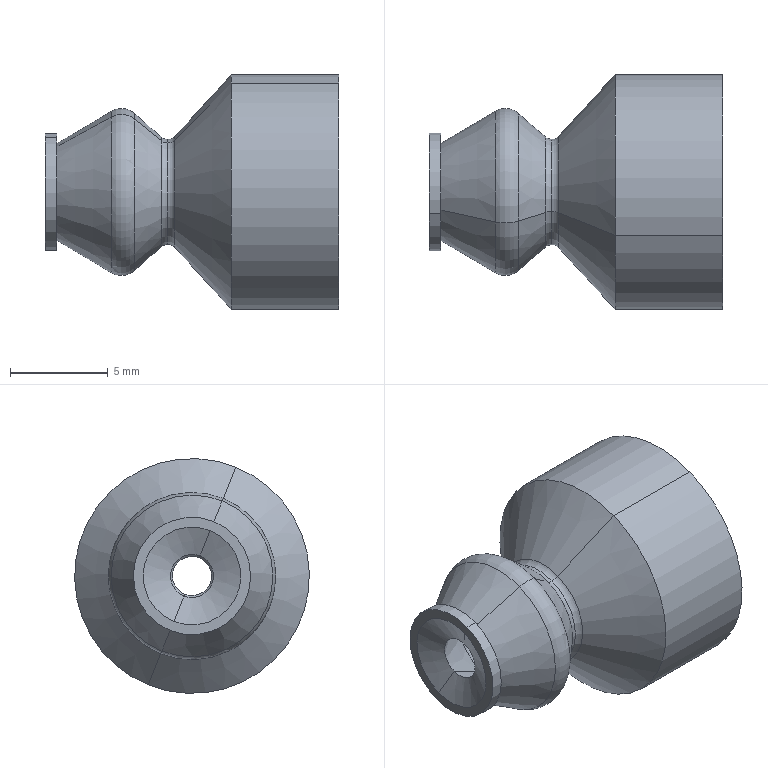Component | SolidWorks | VPDT6-1 | 1 solid | 37 faces | box 15 x 12 x 12 mm | volume 747 mm3 | cone 12 | torus 10 | cylinder 10 | plane 5 | commonest cylinder face diameters 7 x2 5 x2 12 x2 6 x2 2 x2
build123d program:
from build123d import *

# Parameters (mm, degrees)
SKETCH1_R                 = 3.5
SNAPCAVITYCLEARANCE_DEPTH = 0.7


with BuildPart() as part:
    # Sketch1_2 → Revolve1 (revolve)
    with BuildSketch(Plane.XY, mode=Mode.PRIVATE) as revolve1_sk:
        with BuildLine():
            Line((0, 15), (6, 15))
            Line((6, 15), (6, 9.5))
            Line((6, 9.5), (2.86, 6.629))
            ThreePointArc((2.86, 6.629), (2.698, 6.289), (2.82, 5.932))
            Line((2.82, 5.932), (4.028, 4.543))
            ThreePointArc((4.028, 4.543), (4.269, 3.979), (4.135, 3.38))
            Line((4.135, 3.38), (2.5, 0.6))
            Line((2.5, 0.6), (3, 0.6))
            Line((3, 0.6), (3, 0))
            Line((3, 0), (0, 0))
            Line((0, 0), (0, 15))
        make_face()
    revolve(revolve1_sk.sketch.rotate(Axis((0, 0, 0), (0, 1, 0)), 270), axis=Axis((0, 0, 0), (0, 1, 0)))

    # Sketch2 → Cut-Revolve1 (revolve, cut)
    with BuildSketch(Plane.XY, mode=Mode.PRIVATE) as cut_revolve1_sk:
        with BuildLine():
            Line((0, 15), (2.5, 15))
            Line((2.5, 15), (2.5, 12.5))
            Line((2.5, 12.5), (3.5, 12.5))
            ThreePointArc((3.5, 12.5), (4.5, 11.5), (3.5, 10.5))
            Line((3.5, 10.5), (1, 10.5))
            Line((1, 10.5), (1, 6.3))
            Line((1, 6.3), (2.841, 4.607))
            ThreePointArc((2.841, 4.607), (3.159, 3.967), (2.969, 3.278))
            Line((2.969, 3.278), (1.1, 0.6))
            Line((1.1, 0.6), (2.5, 0))
            Line((2.5, 0), (0, 0))
            Line((0, 0), (0, 15))
        make_face()
    revolve(cut_revolve1_sk.sketch.rotate(Axis((0, 0, 0), (0, 1, 0)), 270), axis=Axis((0, 0, 0), (0, 1, 0)), mode=Mode.SUBTRACT)

    # Sketch1 → SnapCavityClearance (cut)
    with BuildSketch(Plane(origin=(0, 10.5, 0), x_dir=(1, 0, 0), z_dir=(0, 1, 0))):
        with Locations(Location((0, 0, 0), (0, 0, 270))):
            Circle(SKETCH1_R)
    extrude(amount=-SNAPCAVITYCLEARANCE_DEPTH, mode=Mode.SUBTRACT)


solid = part.part

# Placed as in the assembly
solid = solid.moved(Location((-186.952, 37.141, -105.536), (0, 0, -90)))
STEP:
#1=COLOUR_RGB('',0.7922,0.8196,0.9333);
#2=FILL_AREA_STYLE_COLOUR('',#1);
#3=FILL_AREA_STYLE('',(#2));
#4=SURFACE_STYLE_FILL_AREA(#3);
#5=SURFACE_SIDE_STYLE('',(#4));
#6=SURFACE_STYLE_USAGE(.BOTH.,#5);
#7=PRESENTATION_STYLE_ASSIGNMENT((#6));
#8=CARTESIAN_POINT('',(-7.099,1.42,-4.05));
#9=VERTEX_POINT('',#8);
#10=CARTESIAN_POINT('',(-7.114,1.423,-4.056));
#11=VERTEX_POINT('',#10);
#12=CARTESIAN_POINT('',(-7.114,1.415,-4.038));
#13=DIRECTION('',(0.,0.9281,0.3723));
#14=DIRECTION('',(0.,-0.3723,0.9281));
#15=AXIS2_PLACEMENT_3D('',#12,#13,#14);
#16=CIRCLE('',#15,0.01969);
#17=EDGE_CURVE('',#9,#11,#16,.T.);
#18=ORIENTED_EDGE('',*,*,#17,.T.);
#19=CARTESIAN_POINT('',(-7.114,1.502,-4.254));
#20=VERTEX_POINT('',#19);
#21=CARTESIAN_POINT('',(-7.114,1.462,-4.155));
#22=DIRECTION('',(1.,-0.,-0.));
#23=DIRECTION('',(0.,1.,0.));
#24=AXIS2_PLACEMENT_3D('',#21,#22,#23);
#25=CIRCLE('',#24,0.1062);
#26=EDGE_CURVE('',#11,#20,#25,.T.);
#27=ORIENTED_EDGE('',*,*,#26,.T.);
#28=CARTESIAN_POINT('',(-7.099,1.504,-4.259));
#29=VERTEX_POINT('',#28);
#30=CARTESIAN_POINT('',(-7.114,1.509,-4.272));
#31=DIRECTION('',(-0.,-0.9281,-0.3723));
#32=DIRECTION('',(0.,0.3723,-0.9281));
#33=AXIS2_PLACEMENT_3D('',#30,#31,#32);
#34=CIRCLE('',#33,0.01969);
#35=EDGE_CURVE('',#29,#20,#34,.T.);
#36=ORIENTED_EDGE('',*,*,#35,.F.);
#37=CARTESIAN_POINT('',(-7.099,1.462,-4.155));
#38=DIRECTION('',(1.,-0.,-0.));
#39=DIRECTION('',(0.,-0.3723,0.9281));
#40=AXIS2_PLACEMENT_3D('',#37,#38,#39);
#41=CIRCLE('',#40,0.1126);
#42=EDGE_CURVE('',#9,#29,#41,.T.);
#43=ORIENTED_EDGE('',*,*,#42,.F.);
#44=EDGE_LOOP('',(#18,#27,#36,#43));
#45=FACE_OUTER_BOUND('',#44,.T.);
#46=CARTESIAN_POINT('',(-7.114,1.462,-4.155));
#47=DIRECTION('',(1.,-0.,-0.));
#48=DIRECTION('',(-0.,-0.3723,0.9281));
#49=AXIS2_PLACEMENT_3D('',#46,#47,#48);
#50=TOROIDAL_SURFACE('',#49,0.1259,0.01969);
#51=ADVANCED_FACE('',(#45),#50,.F.);
#52=ORIENTED_EDGE('',*,*,#35,.T.);
#53=CARTESIAN_POINT('',(-7.114,1.462,-4.155));
#54=DIRECTION('',(1.,-0.,-0.));
#55=DIRECTION('',(0.,1.,0.));
#56=AXIS2_PLACEMENT_3D('',#53,#54,#55);
#57=CIRCLE('',#56,0.1062);
#58=EDGE_CURVE('',#20,#11,#57,.T.);
#59=ORIENTED_EDGE('',*,*,#58,.T.);
#60=ORIENTED_EDGE('',*,*,#17,.F.);
#61=CARTESIAN_POINT('',(-7.099,1.462,-4.155));
#62=DIRECTION('',(1.,-0.,-0.));
#63=DIRECTION('',(0.,-0.3723,0.9281));
#64=AXIS2_PLACEMENT_3D('',#61,#62,#63);
#65=CIRCLE('',#64,0.1126);
#66=EDGE_CURVE('',#29,#9,#65,.T.);
#67=ORIENTED_EDGE('',*,*,#66,.F.);
#68=EDGE_LOOP('',(#52,#59,#60,#67));
#69=FACE_OUTER_BOUND('',#68,.T.);
#70=CARTESIAN_POINT('',(-7.114,1.462,-4.155));
#71=DIRECTION('',(1.,-0.,-0.));
#72=DIRECTION('',(-0.,-0.3723,0.9281));
#73=AXIS2_PLACEMENT_3D('',#70,#71,#72);
#74=TOROIDAL_SURFACE('',#73,0.1259,0.01969);
#75=ADVANCED_FACE('',(#69),#74,.F.);
#76=CARTESIAN_POINT('',(-6.974,1.514,-4.283));
#77=VERTEX_POINT('',#76);
#78=CARTESIAN_POINT('',(-6.974,1.411,-4.027));
#79=VERTEX_POINT('',#78);
#80=CARTESIAN_POINT('',(-6.974,1.462,-4.155));
#81=DIRECTION('',(1.,-0.,-0.));
#82=DIRECTION('',(0.,-0.3723,0.9281));
#83=AXIS2_PLACEMENT_3D('',#80,#81,#82);
#84=CIRCLE('',#83,0.1378);
#85=EDGE_CURVE('',#77,#79,#84,.T.);
#86=ORIENTED_EDGE('',*,*,#85,.F.);
#87=CARTESIAN_POINT('',(-6.947,1.514,-4.283));
#88=VERTEX_POINT('',#87);
#89=CARTESIAN_POINT('',(-6.974,1.514,-4.283));
#90=DIRECTION('',(1.,-0.,-0.));
#91=VECTOR('',#90,39.37);
#92=LINE('',#89,#91);
#93=EDGE_CURVE('',#77,#88,#92,.T.);
#94=ORIENTED_EDGE('',*,*,#93,.T.);
#95=CARTESIAN_POINT('',(-6.947,1.411,-4.027));
#96=VERTEX_POINT('',#95);
#97=CARTESIAN_POINT('',(-6.947,1.462,-4.155));
#98=DIRECTION('',(1.,-0.,-0.));
#99=DIRECTION('',(0.,-0.3723,0.9281));
#100=AXIS2_PLACEMENT_3D('',#97,#98,#99);
#101=CIRCLE('',#100,0.1378);
#102=EDGE_CURVE('',#88,#96,#101,.T.);
#103=ORIENTED_EDGE('',*,*,#102,.T.);
#104=CARTESIAN_POINT('',(-6.974,1.411,-4.027));
#105=DIRECTION('',(1.,-0.,-0.));
#106=VECTOR('',#105,39.37);
#107=LINE('',#104,#106);
#108=EDGE_CURVE('',#79,#96,#107,.T.);
#109=ORIENTED_EDGE('',*,*,#108,.F.);
#110=EDGE_LOOP('',(#86,#94,#103,#109));
#111=FACE_OUTER_BOUND('',#110,.T.);
#112=CARTESIAN_POINT('',(-6.974,1.462,-4.155));
#113=DIRECTION('',(1.,-0.,-0.));
#114=DIRECTION('',(0.,-0.3723,0.9281));
#115=AXIS2_PLACEMENT_3D('',#112,#113,#114);
#116=CYLINDRICAL_SURFACE('',#115,0.1378);
#117=ADVANCED_FACE('',(#111),#116,.F.);
#118=CARTESIAN_POINT('',(-7.337,1.478,-4.195));
#119=VERTEX_POINT('',#118);
#120=CARTESIAN_POINT('',(-7.337,1.446,-4.115));
#121=VERTEX_POINT('',#120);
#122=CARTESIAN_POINT('',(-7.337,1.462,-4.155));
#123=DIRECTION('',(1.,-0.,-0.));
#124=DIRECTION('',(0.,-0.3723,0.9281));
#125=AXIS2_PLACEMENT_3D('',#122,#123,#124);
#126=CIRCLE('',#125,0.04331);
#127=EDGE_CURVE('',#119,#121,#126,.T.);
#128=ORIENTED_EDGE('',*,*,#127,.T.);
#129=CARTESIAN_POINT('',(-7.36,1.426,-4.064));
#130=VERTEX_POINT('',#129);
#131=CARTESIAN_POINT('',(-7.36,1.426,-4.064));
#132=DIRECTION('',(-0.3939,-0.3422,0.8531));
#133=VECTOR('',#132,39.37);
#134=LINE('',#131,#133);
#135=EDGE_CURVE('',#121,#130,#134,.T.);
#136=ORIENTED_EDGE('',*,*,#135,.T.);
#137=CARTESIAN_POINT('',(-7.36,1.499,-4.246));
#138=VERTEX_POINT('',#137);
#139=CARTESIAN_POINT('',(-7.36,1.462,-4.155));
#140=DIRECTION('',(1.,-0.,-0.));
#141=DIRECTION('',(0.,-0.3723,0.9281));
#142=AXIS2_PLACEMENT_3D('',#139,#140,#141);
#143=CIRCLE('',#142,0.09843);
#144=EDGE_CURVE('',#138,#130,#143,.T.);
#145=ORIENTED_EDGE('',*,*,#144,.F.);
#146=CARTESIAN_POINT('',(-7.36,1.499,-4.246));
#147=DIRECTION('',(-0.3939,0.3422,-0.8531));
#148=VECTOR('',#147,39.37);
#149=LINE('',#146,#148);
#150=EDGE_CURVE('',#119,#138,#149,.T.);
#151=ORIENTED_EDGE('',*,*,#150,.F.);
#152=EDGE_LOOP('',(#128,#136,#145,#151));
#153=FACE_OUTER_BOUND('',#152,.T.);
#154=CARTESIAN_POINT('',(-7.36,1.462,-4.155));
#155=DIRECTION('',(-1.,0.,0.));
#156=DIRECTION('',(0.,0.3723,-0.9281));
#157=AXIS2_PLACEMENT_3D('',#154,#155,#156);
#158=CONICAL_SURFACE('',#157,0.09843,1.166);
#159=ADVANCED_FACE('',(#153),#158,.F.);
#160=ORIENTED_EDGE('',*,*,#127,.F.);
#161=CARTESIAN_POINT('',(-7.231,1.506,-4.263));
#162=VERTEX_POINT('',#161);
#163=CARTESIAN_POINT('',(-7.337,1.478,-4.195));
#164=DIRECTION('',(0.82,0.2131,-0.5312));
#165=VECTOR('',#164,39.37);
#166=LINE('',#163,#165);
#167=EDGE_CURVE('',#119,#162,#166,.T.);
#168=ORIENTED_EDGE('',*,*,#167,.T.);
#169=CARTESIAN_POINT('',(-7.231,1.419,-4.046));
#170=VERTEX_POINT('',#169);
#171=CARTESIAN_POINT('',(-7.231,1.462,-4.155));
#172=DIRECTION('',(1.,-0.,-0.));
#173=DIRECTION('',(0.,-0.3723,0.9281));
#174=AXIS2_PLACEMENT_3D('',#171,#172,#173);
#175=CIRCLE('',#174,0.1169);
#176=EDGE_CURVE('',#162,#170,#175,.T.);
#177=ORIENTED_EDGE('',*,*,#176,.T.);
#178=CARTESIAN_POINT('',(-7.337,1.446,-4.115));
#179=DIRECTION('',(0.82,-0.2131,0.5312));
#180=VECTOR('',#179,39.37);
#181=LINE('',#178,#180);
#182=EDGE_CURVE('',#121,#170,#181,.T.);
#183=ORIENTED_EDGE('',*,*,#182,.F.);
#184=EDGE_LOOP('',(#160,#168,#177,#183));
#185=FACE_OUTER_BOUND('',#184,.T.);
#186=CARTESIAN_POINT('',(-7.337,1.462,-4.155));
#187=DIRECTION('',(1.,-0.,-0.));
#188=DIRECTION('',(0.,-0.3723,0.9281));
#189=AXIS2_PLACEMENT_3D('',#186,#187,#188);
#190=CONICAL_SURFACE('',#189,0.04331,0.6094);
#191=ADVANCED_FACE('',(#185),#190,.F.);
#192=ORIENTED_EDGE('',*,*,#176,.F.);
#193=CARTESIAN_POINT('',(-7.179,1.504,-4.259));
#194=VERTEX_POINT('',#193);
#195=CARTESIAN_POINT('',(-7.208,1.494,-4.234));
#196=DIRECTION('',(-0.,-0.9281,-0.3723));
#197=DIRECTION('',(0.,0.3723,-0.9281));
#198=AXIS2_PLACEMENT_3D('',#195,#196,#197);
#199=CIRCLE('',#198,0.03937);
#200=EDGE_CURVE('',#162,#194,#199,.T.);
#201=ORIENTED_EDGE('',*,*,#200,.T.);
#202=CARTESIAN_POINT('',(-7.179,1.421,-4.051));
#203=VERTEX_POINT('',#202);
#204=CARTESIAN_POINT('',(-7.179,1.462,-4.155));
#205=DIRECTION('',(1.,-0.,-0.));
#206=DIRECTION('',(0.,-0.3723,0.9281));
#207=AXIS2_PLACEMENT_3D('',#204,#205,#206);
#208=CIRCLE('',#207,0.1118);
#209=EDGE_CURVE('',#194,#203,#208,.T.);
#210=ORIENTED_EDGE('',*,*,#209,.T.);
#211=CARTESIAN_POINT('',(-7.208,1.431,-4.076));
#212=DIRECTION('',(0.,0.9281,0.3723));
#213=DIRECTION('',(0.,-0.3723,0.9281));
#214=AXIS2_PLACEMENT_3D('',#211,#212,#213);
#215=CIRCLE('',#214,0.03937);
#216=EDGE_CURVE('',#170,#203,#215,.T.);
#217=ORIENTED_EDGE('',*,*,#216,.F.);
#218=EDGE_LOOP('',(#192,#201,#210,#217));
#219=FACE_OUTER_BOUND('',#218,.T.);
#220=CARTESIAN_POINT('',(-7.208,1.462,-4.155));
#221=DIRECTION('',(1.,-0.,-0.));
#222=DIRECTION('',(-0.,-0.3723,0.9281));
#223=AXIS2_PLACEMENT_3D('',#220,#221,#222);
#224=TOROIDAL_SURFACE('',#223,0.08518,0.03937);
#225=ADVANCED_FACE('',(#219),#224,.F.);
#226=CARTESIAN_POINT('',(-7.112,1.477,-4.192));
#227=VERTEX_POINT('',#226);
#228=CARTESIAN_POINT('',(-7.112,1.448,-4.118));
#229=VERTEX_POINT('',#228);
#230=CARTESIAN_POINT('',(-7.112,1.462,-4.155));
#231=DIRECTION('',(1.,-0.,-0.));
#232=DIRECTION('',(0.,-0.3723,0.9281));
#233=AXIS2_PLACEMENT_3D('',#230,#231,#232);
#234=CIRCLE('',#233,0.03937);
#235=EDGE_CURVE('',#227,#229,#234,.T.);
#236=ORIENTED_EDGE('',*,*,#235,.T.);
#237=CARTESIAN_POINT('',(-7.179,1.421,-4.051));
#238=DIRECTION('',(-0.6771,-0.274,0.683));
#239=VECTOR('',#238,39.37);
#240=LINE('',#237,#239);
#241=EDGE_CURVE('',#229,#203,#240,.T.);
#242=ORIENTED_EDGE('',*,*,#241,.T.);
#243=ORIENTED_EDGE('',*,*,#209,.F.);
#244=CARTESIAN_POINT('',(-7.179,1.504,-4.259));
#245=DIRECTION('',(-0.6771,0.274,-0.683));
#246=VECTOR('',#245,39.37);
#247=LINE('',#244,#246);
#248=EDGE_CURVE('',#227,#194,#247,.T.);
#249=ORIENTED_EDGE('',*,*,#248,.F.);
#250=EDGE_LOOP('',(#236,#242,#243,#249));
#251=FACE_OUTER_BOUND('',#250,.T.);
#252=CARTESIAN_POINT('',(-7.179,1.462,-4.155));
#253=DIRECTION('',(-1.,0.,0.));
#254=DIRECTION('',(0.,0.3723,-0.9281));
#255=AXIS2_PLACEMENT_3D('',#252,#253,#254);
#256=CONICAL_SURFACE('',#255,0.1118,0.827);
#257=ADVANCED_FACE('',(#251),#256,.F.);
#258=ORIENTED_EDGE('',*,*,#102,.F.);
#259=CARTESIAN_POINT('',(-6.868,1.514,-4.283));
#260=VERTEX_POINT('',#259);
#261=CARTESIAN_POINT('',(-6.908,1.514,-4.283));
#262=DIRECTION('',(-0.,-0.9281,-0.3723));
#263=DIRECTION('',(0.,0.3723,-0.9281));
#264=AXIS2_PLACEMENT_3D('',#261,#262,#263);
#265=CIRCLE('',#264,0.03937);
#266=EDGE_CURVE('',#88,#260,#265,.T.);
#267=ORIENTED_EDGE('',*,*,#266,.T.);
#268=CARTESIAN_POINT('',(-6.868,1.411,-4.027));
#269=VERTEX_POINT('',#268);
#270=CARTESIAN_POINT('',(-6.868,1.462,-4.155));
#271=DIRECTION('',(1.,-0.,-0.));
#272=DIRECTION('',(0.,-0.3723,0.9281));
#273=AXIS2_PLACEMENT_3D('',#270,#271,#272);
#274=CIRCLE('',#273,0.1378);
#275=EDGE_CURVE('',#260,#269,#274,.T.);
#276=ORIENTED_EDGE('',*,*,#275,.T.);
#277=CARTESIAN_POINT('',(-6.908,1.411,-4.027));
#278=DIRECTION('',(0.,0.9281,0.3723));
#279=DIRECTION('',(0.,-0.3723,0.9281));
#280=AXIS2_PLACEMENT_3D('',#277,#278,#279);
#281=CIRCLE('',#280,0.03937);
#282=EDGE_CURVE('',#96,#269,#281,.T.);
#283=ORIENTED_EDGE('',*,*,#282,.F.);
#284=EDGE_LOOP('',(#258,#267,#276,#283));
#285=FACE_OUTER_BOUND('',#284,.T.);
#286=CARTESIAN_POINT('',(-6.908,1.462,-4.155));
#287=DIRECTION('',(1.,-0.,-0.));
#288=DIRECTION('',(-0.,-0.3723,0.9281));
#289=AXIS2_PLACEMENT_3D('',#286,#287,#288);
#290=TOROIDAL_SURFACE('',#289,0.1378,0.03937);
#291=ADVANCED_FACE('',(#285),#290,.F.);
#292=CARTESIAN_POINT('',(-6.868,1.499,-4.246));
#293=VERTEX_POINT('',#292);
#294=CARTESIAN_POINT('',(-6.868,1.426,-4.064));
#295=VERTEX_POINT('',#294);
#296=CARTESIAN_POINT('',(-6.868,1.462,-4.155));
#297=DIRECTION('',(1.,-0.,-0.));
#298=DIRECTION('',(0.,-0.3723,0.9281));
#299=AXIS2_PLACEMENT_3D('',#296,#297,#298);
#300=CIRCLE('',#299,0.09843);
#301=EDGE_CURVE('',#293,#295,#300,.T.);
#302=ORIENTED_EDGE('',*,*,#301,.F.);
#303=CARTESIAN_POINT('',(-6.77,1.499,-4.246));
#304=VERTEX_POINT('',#303);
#305=CARTESIAN_POINT('',(-7.36,1.499,-4.246));
#306=DIRECTION('',(1.,-0.,-0.));
#307=VECTOR('',#306,39.37);
#308=LINE('',#305,#307);
#309=EDGE_CURVE('',#293,#304,#308,.T.);
#310=ORIENTED_EDGE('',*,*,#309,.T.);
#311=CARTESIAN_POINT('',(-6.77,1.426,-4.064));
#312=VERTEX_POINT('',#311);
#313=CARTESIAN_POINT('',(-6.77,1.462,-4.155));
#314=DIRECTION('',(1.,-0.,-0.));
#315=DIRECTION('',(0.,-0.3723,0.9281));
#316=AXIS2_PLACEMENT_3D('',#313,#314,#315);
#317=CIRCLE('',#316,0.09843);
#318=EDGE_CURVE('',#304,#312,#317,.T.);
#319=ORIENTED_EDGE('',*,*,#318,.T.);
#320=CARTESIAN_POINT('',(-7.36,1.426,-4.064));
#321=DIRECTION('',(1.,-0.,-0.));
#322=VECTOR('',#321,39.37);
#323=LINE('',#320,#322);
#324=EDGE_CURVE('',#295,#312,#323,.T.);
#325=ORIENTED_EDGE('',*,*,#324,.F.);
#326=EDGE_LOOP('',(#302,#310,#319,#325));
#327=FACE_OUTER_BOUND('',#326,.T.);
#328=CARTESIAN_POINT('',(-7.36,1.462,-4.155));
#329=DIRECTION('',(1.,-0.,-0.));
#330=DIRECTION('',(0.,-0.3723,0.9281));
#331=AXIS2_PLACEMENT_3D('',#328,#329,#330);
#332=CYLINDRICAL_SURFACE('',#331,0.09843);
#333=ADVANCED_FACE('',(#327),#332,.F.);
#334=CARTESIAN_POINT('',(-6.986,1.374,-3.936));
#335=VERTEX_POINT('',#334);
#336=CARTESIAN_POINT('',(-6.986,1.55,-4.374));
#337=VERTEX_POINT('',#336);
#338=CARTESIAN_POINT('',(-6.986,1.462,-4.155));
#339=DIRECTION('',(1.,-0.,-0.));
#340=DIRECTION('',(0.,-0.3723,0.9281));
#341=AXIS2_PLACEMENT_3D('',#338,#339,#340);
#342=CIRCLE('',#341,0.2362);
#343=EDGE_CURVE('',#335,#337,#342,.T.);
#344=ORIENTED_EDGE('',*,*,#343,.T.);
#345=CARTESIAN_POINT('',(-6.77,1.55,-4.374));
#346=VERTEX_POINT('',#345);
#347=CARTESIAN_POINT('',(-7.36,1.55,-4.374));
#348=DIRECTION('',(1.,-0.,-0.));
#349=VECTOR('',#348,39.37);
#350=LINE('',#347,#349);
#351=EDGE_CURVE('',#337,#346,#350,.T.);
#352=ORIENTED_EDGE('',*,*,#351,.T.);
#353=CARTESIAN_POINT('',(-6.77,1.374,-3.936));
#354=VERTEX_POINT('',#353);
#355=CARTESIAN_POINT('',(-6.77,1.462,-4.155));
#356=DIRECTION('',(1.,-0.,-0.));
#357=DIRECTION('',(0.,-0.3723,0.9281));
#358=AXIS2_PLACEMENT_3D('',#355,#356,#357);
#359=CIRCLE('',#358,0.2362);
#360=EDGE_CURVE('',#354,#346,#359,.T.);
#361=ORIENTED_EDGE('',*,*,#360,.F.);
#362=CARTESIAN_POINT('',(-7.36,1.374,-3.936));
#363=DIRECTION('',(1.,-0.,-0.));
#364=VECTOR('',#363,39.37);
#365=LINE('',#362,#364);
#366=EDGE_CURVE('',#335,#354,#365,.T.);
#367=ORIENTED_EDGE('',*,*,#366,.F.);
#368=EDGE_LOOP('',(#344,#352,#361,#367));
#369=FACE_OUTER_BOUND('',#368,.T.);
#370=CARTESIAN_POINT('',(-7.36,1.462,-4.155));
#371=DIRECTION('',(1.,-0.,-0.));
#372=DIRECTION('',(0.,-0.3723,0.9281));
#373=AXIS2_PLACEMENT_3D('',#370,#371,#372);
#374=CYLINDRICAL_SURFACE('',#373,0.2362);
#375=ADVANCED_FACE('',(#369),#374,.T.);
#376=ORIENTED_EDGE('',*,*,#42,.T.);
#377=CARTESIAN_POINT('',(-7.099,1.504,-4.259));
#378=DIRECTION('',(0.6748,0.2748,-0.685));
#379=VECTOR('',#378,39.37);
#380=LINE('',#377,#379);
#381=EDGE_CURVE('',#29,#337,#380,.T.);
#382=ORIENTED_EDGE('',*,*,#381,.T.);
#383=ORIENTED_EDGE('',*,*,#343,.F.);
#384=CARTESIAN_POINT('',(-7.099,1.42,-4.05));
#385=DIRECTION('',(0.6748,-0.2748,0.685));
#386=VECTOR('',#385,39.37);
#387=LINE('',#384,#386);
#388=EDGE_CURVE('',#9,#335,#387,.T.);
#389=ORIENTED_EDGE('',*,*,#388,.F.);
#390=EDGE_LOOP('',(#376,#382,#383,#389));
#391=FACE_OUTER_BOUND('',#390,.T.);
#392=CARTESIAN_POINT('',(-7.099,1.462,-4.155));
#393=DIRECTION('',(1.,-0.,-0.));
#394=DIRECTION('',(0.,-0.3723,0.9281));
#395=AXIS2_PLACEMENT_3D('',#392,#393,#394);
#396=CONICAL_SURFACE('',#395,0.1126,0.8301);
#397=ADVANCED_FACE('',(#391),#396,.T.);
#398=ORIENTED_EDGE('',*,*,#58,.F.);
#399=CARTESIAN_POINT('',(-7.127,1.504,-4.258));
#400=VERTEX_POINT('',#399);
#401=CARTESIAN_POINT('',(-7.114,1.509,-4.272));
#402=DIRECTION('',(-0.,-0.9281,-0.3723));
#403=DIRECTION('',(0.,0.3723,-0.9281));
#404=AXIS2_PLACEMENT_3D('',#401,#402,#403);
#405=CIRCLE('',#404,0.01969);
#406=EDGE_CURVE('',#20,#400,#405,.T.);
#407=ORIENTED_EDGE('',*,*,#406,.T.);
#408=CARTESIAN_POINT('',(-7.127,1.421,-4.052));
#409=VERTEX_POINT('',#408);
#410=CARTESIAN_POINT('',(-7.127,1.462,-4.155));
#411=DIRECTION('',(1.,-0.,-0.));
#412=DIRECTION('',(0.,-0.3723,0.9281));
#413=AXIS2_PLACEMENT_3D('',#410,#411,#412);
#414=CIRCLE('',#413,0.111);
#415=EDGE_CURVE('',#400,#409,#414,.T.);
#416=ORIENTED_EDGE('',*,*,#415,.T.);
#417=CARTESIAN_POINT('',(-7.114,1.415,-4.038));
#418=DIRECTION('',(0.,0.9281,0.3723));
#419=DIRECTION('',(0.,-0.3723,0.9281));
#420=AXIS2_PLACEMENT_3D('',#417,#418,#419);
#421=CIRCLE('',#420,0.01969);
#422=EDGE_CURVE('',#11,#409,#421,.T.);
#423=ORIENTED_EDGE('',*,*,#422,.F.);
#424=EDGE_LOOP('',(#398,#407,#416,#423));
#425=FACE_OUTER_BOUND('',#424,.T.);
#426=CARTESIAN_POINT('',(-7.114,1.462,-4.155));
#427=DIRECTION('',(1.,-0.,-0.));
#428=DIRECTION('',(-0.,-0.3723,0.9281));
#429=AXIS2_PLACEMENT_3D('',#426,#427,#428);
#430=TOROIDAL_SURFACE('',#429,0.1259,0.01969);
#431=ADVANCED_FACE('',(#425),#430,.F.);
#432=CARTESIAN_POINT('',(-7.127,1.462,-4.155));
#433=DIRECTION('',(1.,-0.,-0.));
#434=DIRECTION('',(0.,-0.3723,0.9281));
#435=AXIS2_PLACEMENT_3D('',#432,#433,#434);
#436=CIRCLE('',#435,0.111);
#437=EDGE_CURVE('',#409,#400,#436,.T.);
#438=ORIENTED_EDGE('',*,*,#437,.F.);
#439=CARTESIAN_POINT('',(-7.181,1.403,-4.008));
#440=VERTEX_POINT('',#439);
#441=CARTESIAN_POINT('',(-7.181,1.403,-4.008));
#442=DIRECTION('',(-0.7546,-0.2443,0.609));
#443=VECTOR('',#442,39.37);
#444=LINE('',#441,#443);
#445=EDGE_CURVE('',#409,#440,#444,.T.);
#446=ORIENTED_EDGE('',*,*,#445,.T.);
#447=CARTESIAN_POINT('',(-7.181,1.521,-4.302));
#448=VERTEX_POINT('',#447);
#449=CARTESIAN_POINT('',(-7.181,1.462,-4.155));
#450=DIRECTION('',(1.,-0.,-0.));
#451=DIRECTION('',(0.,-0.3723,0.9281));
#452=AXIS2_PLACEMENT_3D('',#449,#450,#451);
#453=CIRCLE('',#452,0.1586);
#454=EDGE_CURVE('',#440,#448,#453,.T.);
#455=ORIENTED_EDGE('',*,*,#454,.T.);
#456=CARTESIAN_POINT('',(-7.181,1.521,-4.302));
#457=DIRECTION('',(-0.7546,0.2443,-0.609));
#458=VECTOR('',#457,39.37);
#459=LINE('',#456,#458);
#460=EDGE_CURVE('',#400,#448,#459,.T.);
#461=ORIENTED_EDGE('',*,*,#460,.F.);
#462=EDGE_LOOP('',(#438,#446,#455,#461));
#463=FACE_OUTER_BOUND('',#462,.T.);
#464=CARTESIAN_POINT('',(-7.181,1.462,-4.155));
#465=DIRECTION('',(-1.,0.,0.));
#466=DIRECTION('',(0.,0.3723,-0.9281));
#467=AXIS2_PLACEMENT_3D('',#464,#465,#466);
#468=CONICAL_SURFACE('',#467,0.1586,0.7157);
#469=ADVANCED_FACE('',(#463),#468,.T.);
#470=CARTESIAN_POINT('',(-7.227,1.402,-4.004));
#471=VERTEX_POINT('',#470);
#472=CARTESIAN_POINT('',(-7.227,1.523,-4.306));
#473=VERTEX_POINT('',#472);
#474=CARTESIAN_POINT('',(-7.227,1.462,-4.155));
#475=DIRECTION('',(1.,-0.,-0.));
#476=DIRECTION('',(0.,-0.3723,0.9281));
#477=AXIS2_PLACEMENT_3D('',#474,#475,#476);
#478=CIRCLE('',#477,0.1628);
#479=EDGE_CURVE('',#471,#473,#478,.T.);
#480=ORIENTED_EDGE('',*,*,#479,.T.);
#481=CARTESIAN_POINT('',(-7.207,1.51,-4.275));
#482=DIRECTION('',(-0.,-0.9281,-0.3723));
#483=DIRECTION('',(0.,0.3723,-0.9281));
#484=AXIS2_PLACEMENT_3D('',#481,#482,#483);
#485=CIRCLE('',#484,0.03937);
#486=EDGE_CURVE('',#473,#448,#485,.T.);
#487=ORIENTED_EDGE('',*,*,#486,.T.);
#488=ORIENTED_EDGE('',*,*,#454,.F.);
#489=CARTESIAN_POINT('',(-7.207,1.414,-4.035));
#490=DIRECTION('',(0.,0.9281,0.3723));
#491=DIRECTION('',(0.,-0.3723,0.9281));
#492=AXIS2_PLACEMENT_3D('',#489,#490,#491);
#493=CIRCLE('',#492,0.03937);
#494=EDGE_CURVE('',#471,#440,#493,.T.);
#495=ORIENTED_EDGE('',*,*,#494,.F.);
#496=EDGE_LOOP('',(#480,#487,#488,#495));
#497=FACE_OUTER_BOUND('',#496,.T.);
#498=CARTESIAN_POINT('',(-7.207,1.462,-4.155));
#499=DIRECTION('',(1.,-0.,-0.));
#500=DIRECTION('',(-0.,-0.3723,0.9281));
#501=AXIS2_PLACEMENT_3D('',#498,#499,#500);
#502=TOROIDAL_SURFACE('',#501,0.1289,0.03937);
#503=ADVANCED_FACE('',(#497),#502,.T.);
#504=CARTESIAN_POINT('',(-7.337,1.426,-4.064));
#505=VERTEX_POINT('',#504);
#506=CARTESIAN_POINT('',(-7.337,1.499,-4.246));
#507=VERTEX_POINT('',#506);
#508=CARTESIAN_POINT('',(-7.337,1.462,-4.155));
#509=DIRECTION('',(1.,-0.,-0.));
#510=DIRECTION('',(0.,-0.3723,0.9281));
#511=AXIS2_PLACEMENT_3D('',#508,#509,#510);
#512=CIRCLE('',#511,0.09843);
#513=EDGE_CURVE('',#505,#507,#512,.T.);
#514=ORIENTED_EDGE('',*,*,#513,.T.);
#515=CARTESIAN_POINT('',(-7.337,1.499,-4.246));
#516=DIRECTION('',(0.8619,0.1888,-0.4706));
#517=VECTOR('',#516,39.37);
#518=LINE('',#515,#517);
#519=EDGE_CURVE('',#507,#473,#518,.T.);
#520=ORIENTED_EDGE('',*,*,#519,.T.);
#521=ORIENTED_EDGE('',*,*,#479,.F.);
#522=CARTESIAN_POINT('',(-7.337,1.426,-4.064));
#523=DIRECTION('',(0.8619,-0.1888,0.4706));
#524=VECTOR('',#523,39.37);
#525=LINE('',#522,#524);
#526=EDGE_CURVE('',#505,#471,#525,.T.);
#527=ORIENTED_EDGE('',*,*,#526,.F.);
#528=EDGE_LOOP('',(#514,#520,#521,#527));
#529=FACE_OUTER_BOUND('',#528,.T.);
#530=CARTESIAN_POINT('',(-7.337,1.462,-4.155));
#531=DIRECTION('',(1.,-0.,-0.));
#532=DIRECTION('',(0.,-0.3723,0.9281));
#533=AXIS2_PLACEMENT_3D('',#530,#531,#532);
#534=CONICAL_SURFACE('',#533,0.09843,0.5317);
#535=ADVANCED_FACE('',(#529),#534,.T.);
#536=CARTESIAN_POINT('',(-7.36,1.418,-4.045));
#537=VERTEX_POINT('',#536);
#538=CARTESIAN_POINT('',(-7.36,1.506,-4.265));
#539=VERTEX_POINT('',#538);
#540=CARTESIAN_POINT('',(-7.36,1.462,-4.155));
#541=DIRECTION('',(1.,-0.,-0.));
#542=DIRECTION('',(0.,-0.3723,0.9281));
#543=AXIS2_PLACEMENT_3D('',#540,#541,#542);
#544=CIRCLE('',#543,0.1181);
#545=EDGE_CURVE('',#537,#539,#544,.T.);
#546=ORIENTED_EDGE('',*,*,#545,.T.);
#547=CARTESIAN_POINT('',(-7.337,1.506,-4.265));
#548=VERTEX_POINT('',#547);
#549=CARTESIAN_POINT('',(-7.36,1.506,-4.265));
#550=DIRECTION('',(1.,-0.,-0.));
#551=VECTOR('',#550,39.37);
#552=LINE('',#549,#551);
#553=EDGE_CURVE('',#539,#548,#552,.T.);
#554=ORIENTED_EDGE('',*,*,#553,.T.);
#555=CARTESIAN_POINT('',(-7.337,1.418,-4.045));
#556=VERTEX_POINT('',#555);
#557=CARTESIAN_POINT('',(-7.337,1.462,-4.155));
#558=DIRECTION('',(1.,-0.,-0.));
#559=DIRECTION('',(0.,-0.3723,0.9281));
#560=AXIS2_PLACEMENT_3D('',#557,#558,#559);
#561=CIRCLE('',#560,0.1181);
#562=EDGE_CURVE('',#556,#548,#561,.T.);
#563=ORIENTED_EDGE('',*,*,#562,.F.);
#564=CARTESIAN_POINT('',(-7.36,1.418,-4.045));
#565=DIRECTION('',(1.,-0.,-0.));
#566=VECTOR('',#565,39.37);
#567=LINE('',#564,#566);
#568=EDGE_CURVE('',#537,#556,#567,.T.);
#569=ORIENTED_EDGE('',*,*,#568,.F.);
#570=EDGE_LOOP('',(#546,#554,#563,#569));
#571=FACE_OUTER_BOUND('',#570,.T.);
#572=CARTESIAN_POINT('',(-7.36,1.462,-4.155));
#573=DIRECTION('',(1.,-0.,-0.));
#574=DIRECTION('',(0.,-0.3723,0.9281));
#575=AXIS2_PLACEMENT_3D('',#572,#573,#574);
#576=CYLINDRICAL_SURFACE('',#575,0.1181);
#577=ADVANCED_FACE('',(#571),#576,.T.);
#578=ORIENTED_EDGE('',*,*,#235,.F.);
#579=CARTESIAN_POINT('',(-6.974,1.477,-4.192));
#580=VERTEX_POINT('',#579);
#581=CARTESIAN_POINT('',(-7.36,1.477,-4.192));
#582=DIRECTION('',(1.,-0.,-0.));
#583=VECTOR('',#582,39.37);
#584=LINE('',#581,#583);
#585=EDGE_CURVE('',#227,#580,#584,.T.);
#586=ORIENTED_EDGE('',*,*,#585,.T.);
#587=CARTESIAN_POINT('',(-6.974,1.448,-4.118));
#588=VERTEX_POINT('',#587);
#589=CARTESIAN_POINT('',(-6.974,1.462,-4.155));
#590=DIRECTION('',(1.,-0.,-0.));
#591=DIRECTION('',(0.,-0.3723,0.9281));
#592=AXIS2_PLACEMENT_3D('',#589,#590,#591);
#593=CIRCLE('',#592,0.03937);
#594=EDGE_CURVE('',#580,#588,#593,.T.);
#595=ORIENTED_EDGE('',*,*,#594,.T.);
#596=CARTESIAN_POINT('',(-7.36,1.448,-4.118));
#597=DIRECTION('',(1.,-0.,-0.));
#598=VECTOR('',#597,39.37);
#599=LINE('',#596,#598);
#600=EDGE_CURVE('',#229,#588,#599,.T.);
#601=ORIENTED_EDGE('',*,*,#600,.F.);
#602=EDGE_LOOP('',(#578,#586,#595,#601));
#603=FACE_OUTER_BOUND('',#602,.T.);
#604=CARTESIAN_POINT('',(-7.36,1.462,-4.155));
#605=DIRECTION('',(1.,-0.,-0.));
#606=DIRECTION('',(0.,-0.3723,0.9281));
#607=AXIS2_PLACEMENT_3D('',#604,#605,#606);
#608=CYLINDRICAL_SURFACE('',#607,0.03937);
#609=ADVANCED_FACE('',(#603),#608,.F.);
#610=ORIENTED_EDGE('',*,*,#585,.F.);
#611=CARTESIAN_POINT('',(-7.112,1.462,-4.155));
#612=DIRECTION('',(1.,-0.,-0.));
#613=DIRECTION('',(0.,-0.3723,0.9281));
#614=AXIS2_PLACEMENT_3D('',#611,#612,#613);
#615=CIRCLE('',#614,0.03937);
#616=EDGE_CURVE('',#229,#227,#615,.T.);
#617=ORIENTED_EDGE('',*,*,#616,.F.);
#618=ORIENTED_EDGE('',*,*,#600,.T.);
#619=CARTESIAN_POINT('',(-6.974,1.462,-4.155));
#620=DIRECTION('',(1.,-0.,-0.));
#621=DIRECTION('',(0.,-0.3723,0.9281));
#622=AXIS2_PLACEMENT_3D('',#619,#620,#621);
#623=CIRCLE('',#622,0.03937);
#624=EDGE_CURVE('',#588,#580,#623,.T.);
#625=ORIENTED_EDGE('',*,*,#624,.T.);
#626=EDGE_LOOP('',(#610,#617,#618,#625));
#627=FACE_OUTER_BOUND('',#626,.T.);
#628=CARTESIAN_POINT('',(-7.36,1.462,-4.155));
#629=DIRECTION('',(1.,-0.,-0.));
#630=DIRECTION('',(0.,-0.3723,0.9281));
#631=AXIS2_PLACEMENT_3D('',#628,#629,#630);
#632=CYLINDRICAL_SURFACE('',#631,0.03937);
#633=ADVANCED_FACE('',(#627),#632,.F.);
#634=ORIENTED_EDGE('',*,*,#545,.F.);
#635=CARTESIAN_POINT('',(-7.36,1.462,-4.155));
#636=DIRECTION('',(1.,-0.,-0.));
#637=DIRECTION('',(0.,-0.3723,0.9281));
#638=AXIS2_PLACEMENT_3D('',#635,#636,#637);
#639=CIRCLE('',#638,0.1181);
#640=EDGE_CURVE('',#539,#537,#639,.T.);
#641=ORIENTED_EDGE('',*,*,#640,.F.);
#642=EDGE_LOOP('',(#634,#641));
#643=FACE_OUTER_BOUND('',#642,.T.);
#644=ORIENTED_EDGE('',*,*,#144,.T.);
#645=CARTESIAN_POINT('',(-7.36,1.462,-4.155));
#646=DIRECTION('',(1.,-0.,-0.));
#647=DIRECTION('',(0.,-0.3723,0.9281));
#648=AXIS2_PLACEMENT_3D('',#645,#646,#647);
#649=CIRCLE('',#648,0.09843);
#650=EDGE_CURVE('',#130,#138,#649,.T.);
#651=ORIENTED_EDGE('',*,*,#650,.T.);
#652=EDGE_LOOP('',(#644,#651));
#653=FACE_BOUND('',#652,.T.);
#654=CARTESIAN_POINT('',(-7.36,1.353,-4.199));
#655=DIRECTION('',(1.,-0.,-0.));
#656=DIRECTION('',(-0.,-0.3723,0.9281));
#657=AXIS2_PLACEMENT_3D('',#654,#655,#656);
#658=PLANE('',#657);
#659=ADVANCED_FACE('',(#643,#653),#658,.F.);
#660=ORIENTED_EDGE('',*,*,#360,.T.);
#661=CARTESIAN_POINT('',(-6.77,1.462,-4.155));
#662=DIRECTION('',(1.,-0.,-0.));
#663=DIRECTION('',(0.,-0.3723,0.9281));
#664=AXIS2_PLACEMENT_3D('',#661,#662,#663);
#665=CIRCLE('',#664,0.2362);
#666=EDGE_CURVE('',#346,#354,#665,.T.);
#667=ORIENTED_EDGE('',*,*,#666,.T.);
#668=EDGE_LOOP('',(#660,#667));
#669=FACE_OUTER_BOUND('',#668,.T.);
#670=CARTESIAN_POINT('',(-6.77,1.462,-4.155));
#671=DIRECTION('',(1.,-0.,-0.));
#672=DIRECTION('',(0.,-0.3723,0.9281));
#673=AXIS2_PLACEMENT_3D('',#670,#671,#672);
#674=CIRCLE('',#673,0.09843);
#675=EDGE_CURVE('',#312,#304,#674,.T.);
#676=ORIENTED_EDGE('',*,*,#675,.F.);
#677=ORIENTED_EDGE('',*,*,#318,.F.);
#678=EDGE_LOOP('',(#676,#677));
#679=FACE_BOUND('',#678,.T.);
#680=CARTESIAN_POINT('',(-6.77,1.462,-4.155));
#681=DIRECTION('',(-1.,0.,0.));
#682=DIRECTION('',(0.,0.3723,-0.9281));
#683=AXIS2_PLACEMENT_3D('',#680,#681,#682);
#684=PLANE('',#683);
#685=ADVANCED_FACE('',(#669,#679),#684,.F.);
#686=ORIENTED_EDGE('',*,*,#553,.F.);
#687=ORIENTED_EDGE('',*,*,#640,.T.);
#688=ORIENTED_EDGE('',*,*,#568,.T.);
#689=CARTESIAN_POINT('',(-7.337,1.462,-4.155));
#690=DIRECTION('',(1.,-0.,-0.));
#691=DIRECTION('',(0.,-0.3723,0.9281));
#692=AXIS2_PLACEMENT_3D('',#689,#690,#691);
#693=CIRCLE('',#692,0.1181);
#694=EDGE_CURVE('',#548,#556,#693,.T.);
#695=ORIENTED_EDGE('',*,*,#694,.F.);
#696=EDGE_LOOP('',(#686,#687,#688,#695));
#697=FACE_OUTER_BOUND('',#696,.T.);
#698=CARTESIAN_POINT('',(-7.36,1.462,-4.155));
#699=DIRECTION('',(1.,-0.,-0.));
#700=DIRECTION('',(0.,-0.3723,0.9281));
#701=AXIS2_PLACEMENT_3D('',#698,#699,#700);
#702=CYLINDRICAL_SURFACE('',#701,0.1181);
#703=ADVANCED_FACE('',(#697),#702,.T.);
#704=ORIENTED_EDGE('',*,*,#513,.F.);
#705=CARTESIAN_POINT('',(-7.337,1.462,-4.155));
#706=DIRECTION('',(1.,-0.,-0.));
#707=DIRECTION('',(0.,-0.3723,0.9281));
#708=AXIS2_PLACEMENT_3D('',#705,#706,#707);
#709=CIRCLE('',#708,0.09843);
#710=EDGE_CURVE('',#507,#505,#709,.T.);
#711=ORIENTED_EDGE('',*,*,#710,.F.);
#712=EDGE_LOOP('',(#704,#711));
#713=FACE_BOUND('',#712,.T.);
#714=ORIENTED_EDGE('',*,*,#562,.T.);
#715=ORIENTED_EDGE('',*,*,#694,.T.);
#716=EDGE_LOOP('',(#714,#715));
#717=FACE_OUTER_BOUND('',#716,.T.);
#718=CARTESIAN_POINT('',(-7.337,1.371,-4.192));
#719=DIRECTION('',(-1.,0.,0.));
#720=DIRECTION('',(0.,0.3723,-0.9281));
#721=AXIS2_PLACEMENT_3D('',#718,#719,#720);
#722=PLANE('',#721);
#723=ADVANCED_FACE('',(#713,#717),#722,.F.);
#724=ORIENTED_EDGE('',*,*,#519,.F.);
#725=ORIENTED_EDGE('',*,*,#710,.T.);
#726=ORIENTED_EDGE('',*,*,#526,.T.);
#727=CARTESIAN_POINT('',(-7.227,1.462,-4.155));
#728=DIRECTION('',(1.,-0.,-0.));
#729=DIRECTION('',(0.,-0.3723,0.9281));
#730=AXIS2_PLACEMENT_3D('',#727,#728,#729);
#731=CIRCLE('',#730,0.1628);
#732=EDGE_CURVE('',#473,#471,#731,.T.);
#733=ORIENTED_EDGE('',*,*,#732,.F.);
#734=EDGE_LOOP('',(#724,#725,#726,#733));
#735=FACE_OUTER_BOUND('',#734,.T.);
#736=CARTESIAN_POINT('',(-7.337,1.462,-4.155));
#737=DIRECTION('',(1.,-0.,-0.));
#738=DIRECTION('',(0.,-0.3723,0.9281));
#739=AXIS2_PLACEMENT_3D('',#736,#737,#738);
#740=CONICAL_SURFACE('',#739,0.09843,0.5317);
#741=ADVANCED_FACE('',(#735),#740,.T.);
#742=ORIENTED_EDGE('',*,*,#486,.F.);
#743=ORIENTED_EDGE('',*,*,#732,.T.);
#744=ORIENTED_EDGE('',*,*,#494,.T.);
#745=CARTESIAN_POINT('',(-7.181,1.462,-4.155));
#746=DIRECTION('',(1.,-0.,-0.));
#747=DIRECTION('',(0.,-0.3723,0.9281));
#748=AXIS2_PLACEMENT_3D('',#745,#746,#747);
#749=CIRCLE('',#748,0.1586);
#750=EDGE_CURVE('',#448,#440,#749,.T.);
#751=ORIENTED_EDGE('',*,*,#750,.F.);
#752=EDGE_LOOP('',(#742,#743,#744,#751));
#753=FACE_OUTER_BOUND('',#752,.T.);
#754=CARTESIAN_POINT('',(-7.207,1.462,-4.155));
#755=DIRECTION('',(1.,-0.,-0.));
#756=DIRECTION('',(-0.,-0.3723,0.9281));
#757=AXIS2_PLACEMENT_3D('',#754,#755,#756);
#758=TOROIDAL_SURFACE('',#757,0.1289,0.03937);
#759=ADVANCED_FACE('',(#753),#758,.T.);
#760=ORIENTED_EDGE('',*,*,#445,.F.);
#761=ORIENTED_EDGE('',*,*,#415,.F.);
#762=ORIENTED_EDGE('',*,*,#460,.T.);
#763=ORIENTED_EDGE('',*,*,#750,.T.);
#764=EDGE_LOOP('',(#760,#761,#762,#763));
#765=FACE_OUTER_BOUND('',#764,.T.);
#766=CARTESIAN_POINT('',(-7.181,1.462,-4.155));
#767=DIRECTION('',(-1.,0.,0.));
#768=DIRECTION('',(0.,0.3723,-0.9281));
#769=AXIS2_PLACEMENT_3D('',#766,#767,#768);
#770=CONICAL_SURFACE('',#769,0.1586,0.7157);
#771=ADVANCED_FACE('',(#765),#770,.T.);
#772=ORIENTED_EDGE('',*,*,#26,.F.);
#773=ORIENTED_EDGE('',*,*,#422,.T.);
#774=ORIENTED_EDGE('',*,*,#437,.T.);
#775=ORIENTED_EDGE('',*,*,#406,.F.);
#776=EDGE_LOOP('',(#772,#773,#774,#775));
#777=FACE_OUTER_BOUND('',#776,.T.);
#778=CARTESIAN_POINT('',(-7.114,1.462,-4.155));
#779=DIRECTION('',(1.,-0.,-0.));
#780=DIRECTION('',(-0.,-0.3723,0.9281));
#781=AXIS2_PLACEMENT_3D('',#778,#779,#780);
#782=TOROIDAL_SURFACE('',#781,0.1259,0.01969);
#783=ADVANCED_FACE('',(#777),#782,.F.);
#784=ORIENTED_EDGE('',*,*,#381,.F.);
#785=ORIENTED_EDGE('',*,*,#66,.T.);
#786=ORIENTED_EDGE('',*,*,#388,.T.);
#787=CARTESIAN_POINT('',(-6.986,1.462,-4.155));
#788=DIRECTION('',(1.,-0.,-0.));
#789=DIRECTION('',(0.,-0.3723,0.9281));
#790=AXIS2_PLACEMENT_3D('',#787,#788,#789);
#791=CIRCLE('',#790,0.2362);
#792=EDGE_CURVE('',#337,#335,#791,.T.);
#793=ORIENTED_EDGE('',*,*,#792,.F.);
#794=EDGE_LOOP('',(#784,#785,#786,#793));
#795=FACE_OUTER_BOUND('',#794,.T.);
#796=CARTESIAN_POINT('',(-7.099,1.462,-4.155));
#797=DIRECTION('',(1.,-0.,-0.));
#798=DIRECTION('',(0.,-0.3723,0.9281));
#799=AXIS2_PLACEMENT_3D('',#796,#797,#798);
#800=CONICAL_SURFACE('',#799,0.1126,0.8301);
#801=ADVANCED_FACE('',(#795),#800,.T.);
#802=ORIENTED_EDGE('',*,*,#351,.F.);
#803=ORIENTED_EDGE('',*,*,#792,.T.);
#804=ORIENTED_EDGE('',*,*,#366,.T.);
#805=ORIENTED_EDGE('',*,*,#666,.F.);
#806=EDGE_LOOP('',(#802,#803,#804,#805));
#807=FACE_OUTER_BOUND('',#806,.T.);
#808=CARTESIAN_POINT('',(-7.36,1.462,-4.155));
#809=DIRECTION('',(1.,-0.,-0.));
#810=DIRECTION('',(0.,-0.3723,0.9281));
#811=AXIS2_PLACEMENT_3D('',#808,#809,#810);
#812=CYLINDRICAL_SURFACE('',#811,0.2362);
#813=ADVANCED_FACE('',(#807),#812,.T.);
#814=ORIENTED_EDGE('',*,*,#309,.F.);
#815=CARTESIAN_POINT('',(-6.868,1.462,-4.155));
#816=DIRECTION('',(1.,-0.,-0.));
#817=DIRECTION('',(0.,-0.3723,0.9281));
#818=AXIS2_PLACEMENT_3D('',#815,#816,#817);
#819=CIRCLE('',#818,0.09843);
#820=EDGE_CURVE('',#295,#293,#819,.T.);
#821=ORIENTED_EDGE('',*,*,#820,.F.);
#822=ORIENTED_EDGE('',*,*,#324,.T.);
#823=ORIENTED_EDGE('',*,*,#675,.T.);
#824=EDGE_LOOP('',(#814,#821,#822,#823));
#825=FACE_OUTER_BOUND('',#824,.T.);
#826=CARTESIAN_POINT('',(-7.36,1.462,-4.155));
#827=DIRECTION('',(1.,-0.,-0.));
#828=DIRECTION('',(0.,-0.3723,0.9281));
#829=AXIS2_PLACEMENT_3D('',#826,#827,#828);
#830=CYLINDRICAL_SURFACE('',#829,0.09843);
#831=ADVANCED_FACE('',(#825),#830,.F.);
#832=ORIENTED_EDGE('',*,*,#820,.T.);
#833=ORIENTED_EDGE('',*,*,#301,.T.);
#834=EDGE_LOOP('',(#832,#833));
#835=FACE_BOUND('',#834,.T.);
#836=CARTESIAN_POINT('',(-6.868,1.462,-4.155));
#837=DIRECTION('',(1.,-0.,-0.));
#838=DIRECTION('',(0.,-0.3723,0.9281));
#839=AXIS2_PLACEMENT_3D('',#836,#837,#838);
#840=CIRCLE('',#839,0.1378);
#841=EDGE_CURVE('',#269,#260,#840,.T.);
#842=ORIENTED_EDGE('',*,*,#841,.F.);
#843=ORIENTED_EDGE('',*,*,#275,.F.);
#844=EDGE_LOOP('',(#842,#843));
#845=FACE_OUTER_BOUND('',#844,.T.);
#846=CARTESIAN_POINT('',(-6.868,1.371,-4.192));
#847=DIRECTION('',(-1.,0.,0.));
#848=DIRECTION('',(0.,0.3723,-0.9281));
#849=AXIS2_PLACEMENT_3D('',#846,#847,#848);
#850=PLANE('',#849);
#851=ADVANCED_FACE('',(#835,#845),#850,.T.);
#852=ORIENTED_EDGE('',*,*,#266,.F.);
#853=CARTESIAN_POINT('',(-6.947,1.462,-4.155));
#854=DIRECTION('',(1.,-0.,-0.));
#855=DIRECTION('',(0.,-0.3723,0.9281));
#856=AXIS2_PLACEMENT_3D('',#853,#854,#855);
#857=CIRCLE('',#856,0.1378);
#858=EDGE_CURVE('',#96,#88,#857,.T.);
#859=ORIENTED_EDGE('',*,*,#858,.F.);
#860=ORIENTED_EDGE('',*,*,#282,.T.);
#861=ORIENTED_EDGE('',*,*,#841,.T.);
#862=EDGE_LOOP('',(#852,#859,#860,#861));
#863=FACE_OUTER_BOUND('',#862,.T.);
#864=CARTESIAN_POINT('',(-6.908,1.462,-4.155));
#865=DIRECTION('',(1.,-0.,-0.));
#866=DIRECTION('',(-0.,-0.3723,0.9281));
#867=AXIS2_PLACEMENT_3D('',#864,#865,#866);
#868=TOROIDAL_SURFACE('',#867,0.1378,0.03937);
#869=ADVANCED_FACE('',(#863),#868,.F.);
#870=ORIENTED_EDGE('',*,*,#241,.F.);
#871=ORIENTED_EDGE('',*,*,#616,.T.);
#872=ORIENTED_EDGE('',*,*,#248,.T.);
#873=CARTESIAN_POINT('',(-7.179,1.462,-4.155));
#874=DIRECTION('',(1.,-0.,-0.));
#875=DIRECTION('',(0.,-0.3723,0.9281));
#876=AXIS2_PLACEMENT_3D('',#873,#874,#875);
#877=CIRCLE('',#876,0.1118);
#878=EDGE_CURVE('',#203,#194,#877,.T.);
#879=ORIENTED_EDGE('',*,*,#878,.F.);
#880=EDGE_LOOP('',(#870,#871,#872,#879));
#881=FACE_OUTER_BOUND('',#880,.T.);
#882=CARTESIAN_POINT('',(-7.179,1.462,-4.155));
#883=DIRECTION('',(-1.,0.,0.));
#884=DIRECTION('',(0.,0.3723,-0.9281));
#885=AXIS2_PLACEMENT_3D('',#882,#883,#884);
#886=CONICAL_SURFACE('',#885,0.1118,0.827);
#887=ADVANCED_FACE('',(#881),#886,.F.);
#888=ORIENTED_EDGE('',*,*,#200,.F.);
#889=CARTESIAN_POINT('',(-7.231,1.462,-4.155));
#890=DIRECTION('',(1.,-0.,-0.));
#891=DIRECTION('',(0.,-0.3723,0.9281));
#892=AXIS2_PLACEMENT_3D('',#889,#890,#891);
#893=CIRCLE('',#892,0.1169);
#894=EDGE_CURVE('',#170,#162,#893,.T.);
#895=ORIENTED_EDGE('',*,*,#894,.F.);
#896=ORIENTED_EDGE('',*,*,#216,.T.);
#897=ORIENTED_EDGE('',*,*,#878,.T.);
#898=EDGE_LOOP('',(#888,#895,#896,#897));
#899=FACE_OUTER_BOUND('',#898,.T.);
#900=CARTESIAN_POINT('',(-7.208,1.462,-4.155));
#901=DIRECTION('',(1.,-0.,-0.));
#902=DIRECTION('',(-0.,-0.3723,0.9281));
#903=AXIS2_PLACEMENT_3D('',#900,#901,#902);
#904=TOROIDAL_SURFACE('',#903,0.08518,0.03937);
#905=ADVANCED_FACE('',(#899),#904,.F.);
#906=ORIENTED_EDGE('',*,*,#167,.F.);
#907=CARTESIAN_POINT('',(-7.337,1.462,-4.155));
#908=DIRECTION('',(1.,-0.,-0.));
#909=DIRECTION('',(0.,-0.3723,0.9281));
#910=AXIS2_PLACEMENT_3D('',#907,#908,#909);
#911=CIRCLE('',#910,0.04331);
#912=EDGE_CURVE('',#121,#119,#911,.T.);
#913=ORIENTED_EDGE('',*,*,#912,.F.);
#914=ORIENTED_EDGE('',*,*,#182,.T.);
#915=ORIENTED_EDGE('',*,*,#894,.T.);
#916=EDGE_LOOP('',(#906,#913,#914,#915));
#917=FACE_OUTER_BOUND('',#916,.T.);
#918=CARTESIAN_POINT('',(-7.337,1.462,-4.155));
#919=DIRECTION('',(1.,-0.,-0.));
#920=DIRECTION('',(0.,-0.3723,0.9281));
#921=AXIS2_PLACEMENT_3D('',#918,#919,#920);
#922=CONICAL_SURFACE('',#921,0.04331,0.6094);
#923=ADVANCED_FACE('',(#917),#922,.F.);
#924=ORIENTED_EDGE('',*,*,#135,.F.);
#925=ORIENTED_EDGE('',*,*,#912,.T.);
#926=ORIENTED_EDGE('',*,*,#150,.T.);
#927=ORIENTED_EDGE('',*,*,#650,.F.);
#928=EDGE_LOOP('',(#924,#925,#926,#927));
#929=FACE_OUTER_BOUND('',#928,.T.);
#930=CARTESIAN_POINT('',(-7.36,1.462,-4.155));
#931=DIRECTION('',(-1.,0.,0.));
#932=DIRECTION('',(0.,0.3723,-0.9281));
#933=AXIS2_PLACEMENT_3D('',#930,#931,#932);
#934=CONICAL_SURFACE('',#933,0.09843,1.166);
#935=ADVANCED_FACE('',(#929),#934,.F.);
#936=ORIENTED_EDGE('',*,*,#93,.F.);
#937=CARTESIAN_POINT('',(-6.974,1.462,-4.155));
#938=DIRECTION('',(1.,-0.,-0.));
#939=DIRECTION('',(0.,-0.3723,0.9281));
#940=AXIS2_PLACEMENT_3D('',#937,#938,#939);
#941=CIRCLE('',#940,0.1378);
#942=EDGE_CURVE('',#79,#77,#941,.T.);
#943=ORIENTED_EDGE('',*,*,#942,.F.);
#944=ORIENTED_EDGE('',*,*,#108,.T.);
#945=ORIENTED_EDGE('',*,*,#858,.T.);
#946=EDGE_LOOP('',(#936,#943,#944,#945));
#947=FACE_OUTER_BOUND('',#946,.T.);
#948=CARTESIAN_POINT('',(-6.974,1.462,-4.155));
#949=DIRECTION('',(1.,-0.,-0.));
#950=DIRECTION('',(0.,-0.3723,0.9281));
#951=AXIS2_PLACEMENT_3D('',#948,#949,#950);
#952=CYLINDRICAL_SURFACE('',#951,0.1378);
#953=ADVANCED_FACE('',(#947),#952,.F.);
#954=ORIENTED_EDGE('',*,*,#624,.F.);
#955=ORIENTED_EDGE('',*,*,#594,.F.);
#956=EDGE_LOOP('',(#954,#955));
#957=FACE_BOUND('',#956,.T.);
#958=ORIENTED_EDGE('',*,*,#942,.T.);
#959=ORIENTED_EDGE('',*,*,#85,.T.);
#960=EDGE_LOOP('',(#958,#959));
#961=FACE_OUTER_BOUND('',#960,.T.);
#962=CARTESIAN_POINT('',(-6.974,1.462,-4.155));
#963=DIRECTION('',(1.,-0.,-0.));
#964=DIRECTION('',(-0.,-0.3723,0.9281));
#965=AXIS2_PLACEMENT_3D('',#962,#963,#964);
#966=PLANE('',#965);
#967=ADVANCED_FACE('',(#957,#961),#966,.T.);
#968=CLOSED_SHELL('',(#51,#75,#117,#159,#191,#225,#257,#291,#333,#375,#397,#431,#469,#503,#535,#577,#609,#633,#659,#685,#703,#723,#741,#759,#771,#783,#801,#813,#831,#851,#869,#887,#905,#923,#935,#953,#967));
#969=MANIFOLD_SOLID_BREP('',#968);
#970=STYLED_ITEM('',(#7),#969);
#971=(LENGTH_UNIT()NAMED_UNIT(*)SI_UNIT($,.METRE.));
#972=LENGTH_MEASURE_WITH_UNIT(LENGTH_MEASURE(0.0254),#971);
#973=DIMENSIONAL_EXPONENTS(1.,0.,0.,0.,0.,0.,0.);
#974=(CONVERSION_BASED_UNIT('',#972)LENGTH_UNIT()NAMED_UNIT(#973));
#975=UNCERTAINTY_MEASURE_WITH_UNIT(LENGTH_MEASURE(0.00001),#974,'','');
#976=(NAMED_UNIT(*)PLANE_ANGLE_UNIT()SI_UNIT($,.RADIAN.));
#977=(NAMED_UNIT(*)SI_UNIT($,.STERADIAN.)SOLID_ANGLE_UNIT());
#978=(GEOMETRIC_REPRESENTATION_CONTEXT(3)GLOBAL_UNCERTAINTY_ASSIGNED_CONTEXT((#975))GLOBAL_UNIT_ASSIGNED_CONTEXT((#974,#976,#977))REPRESENTATION_CONTEXT('',''));
#979=MECHANICAL_DESIGN_GEOMETRIC_PRESENTATION_REPRESENTATION('',(#970),#978);
#980=PRESENTATION_LAYER_ASSIGNMENT('','',(#970));
#981=CARTESIAN_POINT('',(0.,0.,0.));
#982=DIRECTION('',(0.,0.,1.));
#983=DIRECTION('',(1.,0.,0.));
#984=AXIS2_PLACEMENT_3D('',#981,#982,#983);
#985=(LENGTH_UNIT()NAMED_UNIT(*)SI_UNIT($,.METRE.));
#986=LENGTH_MEASURE_WITH_UNIT(LENGTH_MEASURE(0.0254),#985);
#987=DIMENSIONAL_EXPONENTS(1.,0.,0.,0.,0.,0.,0.);
#988=(CONVERSION_BASED_UNIT('',#986)LENGTH_UNIT()NAMED_UNIT(#987));
#989=UNCERTAINTY_MEASURE_WITH_UNIT(LENGTH_MEASURE(0.00001),#988,'','');
#990=(NAMED_UNIT(*)PLANE_ANGLE_UNIT()SI_UNIT($,.RADIAN.));
#991=(NAMED_UNIT(*)SI_UNIT($,.STERADIAN.)SOLID_ANGLE_UNIT());
#992=(GEOMETRIC_REPRESENTATION_CONTEXT(3)GLOBAL_UNCERTAINTY_ASSIGNED_CONTEXT((#989))GLOBAL_UNIT_ASSIGNED_CONTEXT((#988,#990,#991))REPRESENTATION_CONTEXT('',''));
#993=ADVANCED_BREP_SHAPE_REPRESENTATION('',(#969,#984),#992);